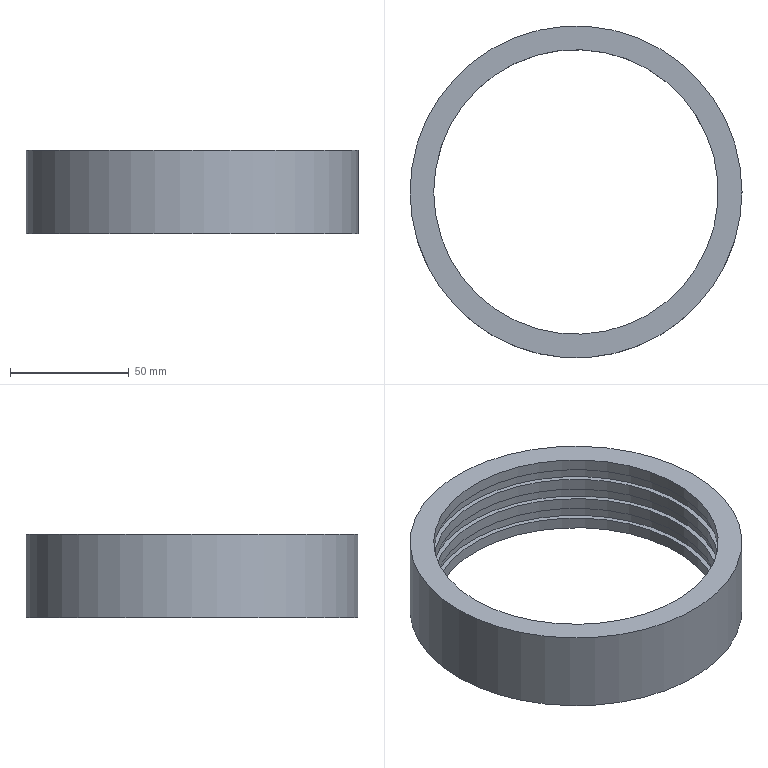Component | NX | CH3404-7 | 1 solid | 16 faces | box 140 x 140 x 35 mm | volume 131444 mm3 | cylinder 8 | plane 8 | commonest cylinder face diameters 120 x4 124 x3 140 x1
STEP:
#1=CARTESIAN_POINT('',(0.,0.,0.));
#2=DIRECTION('',(0.,0.,1.));
#3=DIRECTION('',(1.,0.,0.));
#4=AXIS2_PLACEMENT_3D('',#1,#2,#3);
#5=CARTESIAN_POINT('',(-69.469,0.1057,-1470.003));
#6=VERTEX_POINT('',#5);
#7=CARTESIAN_POINT('',(0.5308,0.1057,-1470.003));
#8=DIRECTION('',(0.,0.,-1.));
#9=DIRECTION('',(-1.,0.,0.));
#10=AXIS2_PLACEMENT_3D('',#7,#8,#9);
#11=CIRCLE('',#10,70.);
#12=CARTESIAN_POINT('',(0.5308,0.1057,-1470.003));
#13=DIRECTION('',(0.,0.,-1.));
#14=DIRECTION('',(-1.,0.,0.));
#15=AXIS2_PLACEMENT_3D('',#12,#13,#14);
#16=CYLINDRICAL_SURFACE('',#15,70.);
#17=CARTESIAN_POINT('',(0.,0.));
#18=DIRECTION('',(1.,0.));
#19=VECTOR('',#18,1.);
#20=LINE('',#17,#19);
#21=(GEOMETRIC_REPRESENTATION_CONTEXT(2)PARAMETRIC_REPRESENTATION_CONTEXT()REPRESENTATION_CONTEXT('',''));
#22=DEFINITIONAL_REPRESENTATION('',(#20),#21);
#23=PCURVE('',#16,#22);
#24=CARTESIAN_POINT('',(0.5308,-69.894,-1470.003));
#25=DIRECTION('',(0.,0.,1.));
#26=DIRECTION('',(1.,0.,0.));
#27=AXIS2_PLACEMENT_3D('',#24,#25,#26);
#28=PLANE('',#27);
#29=CARTESIAN_POINT('',(-70.,70.));
#30=CARTESIAN_POINT('',(-70.,191.244));
#31=CARTESIAN_POINT('',(35.,130.622));
#32=CARTESIAN_POINT('',(140.,70.));
#33=CARTESIAN_POINT('',(35.,9.378));
#34=CARTESIAN_POINT('',(-70.,-51.244));
#35=CARTESIAN_POINT('',(-70.,70.));
#36=(BOUNDED_CURVE()B_SPLINE_CURVE(2,(#29,#30,#31,#32,#33,#34,#35),.UNSPECIFIED.,.T.,.F.)B_SPLINE_CURVE_WITH_KNOTS((1,2,2,2,2,1),(-2.094,0.,2.094,4.189,6.283,8.378),.UNSPECIFIED.)CURVE()GEOMETRIC_REPRESENTATION_ITEM()RATIONAL_B_SPLINE_CURVE((1.,0.5,1.,0.5,1.,0.5,1.))REPRESENTATION_ITEM(''));
#37=(GEOMETRIC_REPRESENTATION_CONTEXT(2)PARAMETRIC_REPRESENTATION_CONTEXT()REPRESENTATION_CONTEXT('',''));
#38=DEFINITIONAL_REPRESENTATION('',(#36),#37);
#39=PCURVE('',#28,#38);
#40=SURFACE_CURVE('',#11,(#23,#39),.PCURVE_S1.);
#41=EDGE_CURVE('',#6,#6,#40,.T.);
#42=ORIENTED_EDGE('',*,*,#41,.F.);
#43=CARTESIAN_POINT('',(-69.469,0.1057,-1435.003));
#44=VERTEX_POINT('',#43);
#45=CARTESIAN_POINT('',(-69.469,0.1057,-1435.003));
#46=CARTESIAN_POINT('',(-69.469,0.1057,-1470.003));
#47=B_SPLINE_CURVE_WITH_KNOTS('',1,(#45,#46),.UNSPECIFIED.,.F.,.F.,(2,2),(-35.,0.),.PIECEWISE_BEZIER_KNOTS.);
#48=CARTESIAN_POINT('',(0.,0.));
#49=DIRECTION('',(0.,1.));
#50=VECTOR('',#49,1.);
#51=LINE('',#48,#50);
#52=(GEOMETRIC_REPRESENTATION_CONTEXT(2)PARAMETRIC_REPRESENTATION_CONTEXT()REPRESENTATION_CONTEXT('',''));
#53=DEFINITIONAL_REPRESENTATION('',(#51),#52);
#54=PCURVE('',#16,#53);
#55=CARTESIAN_POINT('',(6.283,0.));
#56=DIRECTION('',(0.,1.));
#57=VECTOR('',#56,1.);
#58=LINE('',#55,#57);
#59=(GEOMETRIC_REPRESENTATION_CONTEXT(2)PARAMETRIC_REPRESENTATION_CONTEXT()REPRESENTATION_CONTEXT('',''));
#60=DEFINITIONAL_REPRESENTATION('',(#58),#59);
#61=PCURVE('',#16,#60);
#62=SEAM_CURVE('',#47,(#54,#61),.PCURVE_S1.);
#63=EDGE_CURVE('',#44,#6,#62,.T.);
#64=ORIENTED_EDGE('',*,*,#63,.F.);
#65=CARTESIAN_POINT('',(0.5308,0.1057,-1435.003));
#66=DIRECTION('',(0.,0.,-1.));
#67=DIRECTION('',(-1.,0.,0.));
#68=AXIS2_PLACEMENT_3D('',#65,#66,#67);
#69=CIRCLE('',#68,70.);
#70=CARTESIAN_POINT('',(0.,-35.));
#71=DIRECTION('',(1.,0.));
#72=VECTOR('',#71,1.);
#73=LINE('',#70,#72);
#74=(GEOMETRIC_REPRESENTATION_CONTEXT(2)PARAMETRIC_REPRESENTATION_CONTEXT()REPRESENTATION_CONTEXT('',''));
#75=DEFINITIONAL_REPRESENTATION('',(#73),#74);
#76=PCURVE('',#16,#75);
#77=CARTESIAN_POINT('',(0.5308,-59.894,-1435.003));
#78=DIRECTION('',(0.,0.,-1.));
#79=DIRECTION('',(-1.,0.,0.));
#80=AXIS2_PLACEMENT_3D('',#77,#78,#79);
#81=PLANE('',#80);
#82=CARTESIAN_POINT('',(0.,60.));
#83=DIRECTION('',(1.,0.));
#84=AXIS2_PLACEMENT_2D('',#82,#83);
#85=CIRCLE('',#84,70.);
#86=(GEOMETRIC_REPRESENTATION_CONTEXT(2)PARAMETRIC_REPRESENTATION_CONTEXT()REPRESENTATION_CONTEXT('',''));
#87=DEFINITIONAL_REPRESENTATION('',(#85),#86);
#88=PCURVE('',#81,#87);
#89=SURFACE_CURVE('',#69,(#76,#88),.PCURVE_S1.);
#90=EDGE_CURVE('',#44,#44,#89,.T.);
#91=ORIENTED_EDGE('',*,*,#90,.T.);
#92=ORIENTED_EDGE('',*,*,#63,.T.);
#93=EDGE_LOOP('',(#42,#64,#91,#92));
#94=FACE_BOUND('',#93,.T.);
#95=ADVANCED_FACE('',(#94),#16,.T.);
#96=CARTESIAN_POINT('',(-59.469,0.1057,-1470.003));
#97=VERTEX_POINT('',#96);
#98=CARTESIAN_POINT('',(0.5308,0.1057,-1470.003));
#99=DIRECTION('',(0.,0.,-1.));
#100=DIRECTION('',(-1.,0.,0.));
#101=AXIS2_PLACEMENT_3D('',#98,#99,#100);
#102=CIRCLE('',#101,60.);
#103=CARTESIAN_POINT('',(-60.,70.));
#104=CARTESIAN_POINT('',(-60.,173.923));
#105=CARTESIAN_POINT('',(30.,121.962));
#106=CARTESIAN_POINT('',(120.,70.));
#107=CARTESIAN_POINT('',(30.,18.038));
#108=CARTESIAN_POINT('',(-60.,-33.923));
#109=CARTESIAN_POINT('',(-60.,70.));
#110=(BOUNDED_CURVE()B_SPLINE_CURVE(2,(#103,#104,#105,#106,#107,#108,#109),.UNSPECIFIED.,.T.,.F.)B_SPLINE_CURVE_WITH_KNOTS((1,2,2,2,2,1),(-2.094,0.,2.094,4.189,6.283,8.378),.UNSPECIFIED.)CURVE()GEOMETRIC_REPRESENTATION_ITEM()RATIONAL_B_SPLINE_CURVE((1.,0.5,1.,0.5,1.,0.5,1.))REPRESENTATION_ITEM(''));
#111=(GEOMETRIC_REPRESENTATION_CONTEXT(2)PARAMETRIC_REPRESENTATION_CONTEXT()REPRESENTATION_CONTEXT('',''));
#112=DEFINITIONAL_REPRESENTATION('',(#110),#111);
#113=PCURVE('',#28,#112);
#114=CARTESIAN_POINT('',(0.5308,0.1057,-1470.003));
#115=DIRECTION('',(0.,0.,-1.));
#116=DIRECTION('',(-1.,0.,0.));
#117=AXIS2_PLACEMENT_3D('',#114,#115,#116);
#118=CYLINDRICAL_SURFACE('',#117,60.);
#119=CARTESIAN_POINT('',(0.,0.));
#120=DIRECTION('',(1.,0.));
#121=VECTOR('',#120,1.);
#122=LINE('',#119,#121);
#123=(GEOMETRIC_REPRESENTATION_CONTEXT(2)PARAMETRIC_REPRESENTATION_CONTEXT()REPRESENTATION_CONTEXT('',''));
#124=DEFINITIONAL_REPRESENTATION('',(#122),#123);
#125=PCURVE('',#118,#124);
#126=SURFACE_CURVE('',#102,(#113,#125),.PCURVE_S1.);
#127=EDGE_CURVE('',#97,#97,#126,.T.);
#128=ORIENTED_EDGE('',*,*,#127,.F.);
#129=EDGE_LOOP('',(#128));
#130=FACE_BOUND('',#129,.T.);
#131=ORIENTED_EDGE('',*,*,#41,.T.);
#132=EDGE_LOOP('',(#131));
#133=FACE_BOUND('',#132,.T.);
#134=ADVANCED_FACE('',(#130,#133),#28,.F.);
#135=CARTESIAN_POINT('',(-59.469,0.1057,-1465.003));
#136=VERTEX_POINT('',#135);
#137=CARTESIAN_POINT('',(0.5308,0.1057,-1465.003));
#138=DIRECTION('',(0.,0.,-1.));
#139=DIRECTION('',(-1.,0.,0.));
#140=AXIS2_PLACEMENT_3D('',#137,#138,#139);
#141=CIRCLE('',#140,60.);
#142=CARTESIAN_POINT('',(0.,-5.));
#143=DIRECTION('',(1.,0.));
#144=VECTOR('',#143,1.);
#145=LINE('',#142,#144);
#146=(GEOMETRIC_REPRESENTATION_CONTEXT(2)PARAMETRIC_REPRESENTATION_CONTEXT()REPRESENTATION_CONTEXT('',''));
#147=DEFINITIONAL_REPRESENTATION('',(#145),#146);
#148=PCURVE('',#118,#147);
#149=CARTESIAN_POINT('',(0.5308,-59.894,-1465.003));
#150=DIRECTION('',(0.,0.,-1.));
#151=DIRECTION('',(-1.,0.,0.));
#152=AXIS2_PLACEMENT_3D('',#149,#150,#151);
#153=PLANE('',#152);
#154=CARTESIAN_POINT('',(0.,60.));
#155=DIRECTION('',(1.,0.));
#156=AXIS2_PLACEMENT_2D('',#154,#155);
#157=CIRCLE('',#156,60.);
#158=(GEOMETRIC_REPRESENTATION_CONTEXT(2)PARAMETRIC_REPRESENTATION_CONTEXT()REPRESENTATION_CONTEXT('',''));
#159=DEFINITIONAL_REPRESENTATION('',(#157),#158);
#160=PCURVE('',#153,#159);
#161=SURFACE_CURVE('',#141,(#148,#160),.PCURVE_S1.);
#162=EDGE_CURVE('',#136,#136,#161,.T.);
#163=ORIENTED_EDGE('',*,*,#162,.T.);
#164=CARTESIAN_POINT('',(-59.469,0.1057,-1465.003));
#165=CARTESIAN_POINT('',(-59.469,0.1057,-1470.003));
#166=B_SPLINE_CURVE_WITH_KNOTS('',1,(#164,#165),.UNSPECIFIED.,.F.,.F.,(2,2),(-5.,0.),.PIECEWISE_BEZIER_KNOTS.);
#167=CARTESIAN_POINT('',(6.283,0.));
#168=DIRECTION('',(0.,1.));
#169=VECTOR('',#168,1.);
#170=LINE('',#167,#169);
#171=(GEOMETRIC_REPRESENTATION_CONTEXT(2)PARAMETRIC_REPRESENTATION_CONTEXT()REPRESENTATION_CONTEXT('',''));
#172=DEFINITIONAL_REPRESENTATION('',(#170),#171);
#173=PCURVE('',#118,#172);
#174=CARTESIAN_POINT('',(0.,0.));
#175=DIRECTION('',(0.,1.));
#176=VECTOR('',#175,1.);
#177=LINE('',#174,#176);
#178=(GEOMETRIC_REPRESENTATION_CONTEXT(2)PARAMETRIC_REPRESENTATION_CONTEXT()REPRESENTATION_CONTEXT('',''));
#179=DEFINITIONAL_REPRESENTATION('',(#177),#178);
#180=PCURVE('',#118,#179);
#181=SEAM_CURVE('',#166,(#173,#180),.PCURVE_S1.);
#182=EDGE_CURVE('',#136,#97,#181,.T.);
#183=ORIENTED_EDGE('',*,*,#182,.T.);
#184=ORIENTED_EDGE('',*,*,#127,.F.);
#185=ORIENTED_EDGE('',*,*,#182,.F.);
#186=EDGE_LOOP('',(#163,#183,#184,#185));
#187=FACE_BOUND('',#186,.F.);
#188=ADVANCED_FACE('',(#187),#118,.F.);
#189=CARTESIAN_POINT('',(-61.469,0.1057,-1465.003));
#190=VERTEX_POINT('',#189);
#191=CARTESIAN_POINT('',(0.5308,0.1057,-1465.003));
#192=DIRECTION('',(0.,0.,-1.));
#193=DIRECTION('',(-1.,0.,0.));
#194=AXIS2_PLACEMENT_3D('',#191,#192,#193);
#195=CIRCLE('',#194,62.);
#196=CARTESIAN_POINT('',(0.,60.));
#197=DIRECTION('',(1.,0.));
#198=AXIS2_PLACEMENT_2D('',#196,#197);
#199=CIRCLE('',#198,62.);
#200=(GEOMETRIC_REPRESENTATION_CONTEXT(2)PARAMETRIC_REPRESENTATION_CONTEXT()REPRESENTATION_CONTEXT('',''));
#201=DEFINITIONAL_REPRESENTATION('',(#199),#200);
#202=PCURVE('',#153,#201);
#203=CARTESIAN_POINT('',(0.5308,0.1057,-1470.003));
#204=DIRECTION('',(0.,0.,-1.));
#205=DIRECTION('',(-1.,0.,0.));
#206=AXIS2_PLACEMENT_3D('',#203,#204,#205);
#207=CYLINDRICAL_SURFACE('',#206,62.);
#208=CARTESIAN_POINT('',(0.,-5.));
#209=DIRECTION('',(1.,0.));
#210=VECTOR('',#209,1.);
#211=LINE('',#208,#210);
#212=(GEOMETRIC_REPRESENTATION_CONTEXT(2)PARAMETRIC_REPRESENTATION_CONTEXT()REPRESENTATION_CONTEXT('',''));
#213=DEFINITIONAL_REPRESENTATION('',(#211),#212);
#214=PCURVE('',#207,#213);
#215=SURFACE_CURVE('',#195,(#202,#214),.PCURVE_S1.);
#216=EDGE_CURVE('',#190,#190,#215,.T.);
#217=ORIENTED_EDGE('',*,*,#216,.F.);
#218=EDGE_LOOP('',(#217));
#219=FACE_BOUND('',#218,.T.);
#220=ORIENTED_EDGE('',*,*,#162,.T.);
#221=EDGE_LOOP('',(#220));
#222=FACE_BOUND('',#221,.T.);
#223=ADVANCED_FACE('',(#219,#222),#153,.F.);
#224=CARTESIAN_POINT('',(-61.469,0.1057,-1460.003));
#225=VERTEX_POINT('',#224);
#226=CARTESIAN_POINT('',(0.5308,0.1057,-1460.003));
#227=DIRECTION('',(0.,0.,-1.));
#228=DIRECTION('',(-1.,0.,0.));
#229=AXIS2_PLACEMENT_3D('',#226,#227,#228);
#230=CIRCLE('',#229,62.);
#231=CARTESIAN_POINT('',(0.,-10.));
#232=DIRECTION('',(1.,0.));
#233=VECTOR('',#232,1.);
#234=LINE('',#231,#233);
#235=(GEOMETRIC_REPRESENTATION_CONTEXT(2)PARAMETRIC_REPRESENTATION_CONTEXT()REPRESENTATION_CONTEXT('',''));
#236=DEFINITIONAL_REPRESENTATION('',(#234),#235);
#237=PCURVE('',#207,#236);
#238=CARTESIAN_POINT('',(0.5308,-61.894,-1460.003));
#239=DIRECTION('',(0.,0.,1.));
#240=DIRECTION('',(1.,0.,0.));
#241=AXIS2_PLACEMENT_3D('',#238,#239,#240);
#242=PLANE('',#241);
#243=CARTESIAN_POINT('',(-62.,62.));
#244=CARTESIAN_POINT('',(-62.,169.387));
#245=CARTESIAN_POINT('',(31.,115.694));
#246=CARTESIAN_POINT('',(124.,62.));
#247=CARTESIAN_POINT('',(31.,8.306));
#248=CARTESIAN_POINT('',(-62.,-45.387));
#249=CARTESIAN_POINT('',(-62.,62.));
#250=(BOUNDED_CURVE()B_SPLINE_CURVE(2,(#243,#244,#245,#246,#247,#248,#249),.UNSPECIFIED.,.T.,.F.)B_SPLINE_CURVE_WITH_KNOTS((1,2,2,2,2,1),(-2.094,0.,2.094,4.189,6.283,8.378),.UNSPECIFIED.)CURVE()GEOMETRIC_REPRESENTATION_ITEM()RATIONAL_B_SPLINE_CURVE((1.,0.5,1.,0.5,1.,0.5,1.))REPRESENTATION_ITEM(''));
#251=(GEOMETRIC_REPRESENTATION_CONTEXT(2)PARAMETRIC_REPRESENTATION_CONTEXT()REPRESENTATION_CONTEXT('',''));
#252=DEFINITIONAL_REPRESENTATION('',(#250),#251);
#253=PCURVE('',#242,#252);
#254=SURFACE_CURVE('',#230,(#237,#253),.PCURVE_S1.);
#255=EDGE_CURVE('',#225,#225,#254,.T.);
#256=ORIENTED_EDGE('',*,*,#255,.T.);
#257=CARTESIAN_POINT('',(-61.469,0.1057,-1460.003));
#258=CARTESIAN_POINT('',(-61.469,0.1057,-1465.003));
#259=B_SPLINE_CURVE_WITH_KNOTS('',1,(#257,#258),.UNSPECIFIED.,.F.,.F.,(2,2),(-10.,-5.),.PIECEWISE_BEZIER_KNOTS.);
#260=CARTESIAN_POINT('',(6.283,0.));
#261=DIRECTION('',(0.,1.));
#262=VECTOR('',#261,1.);
#263=LINE('',#260,#262);
#264=(GEOMETRIC_REPRESENTATION_CONTEXT(2)PARAMETRIC_REPRESENTATION_CONTEXT()REPRESENTATION_CONTEXT('',''));
#265=DEFINITIONAL_REPRESENTATION('',(#263),#264);
#266=PCURVE('',#207,#265);
#267=CARTESIAN_POINT('',(0.,0.));
#268=DIRECTION('',(0.,1.));
#269=VECTOR('',#268,1.);
#270=LINE('',#267,#269);
#271=(GEOMETRIC_REPRESENTATION_CONTEXT(2)PARAMETRIC_REPRESENTATION_CONTEXT()REPRESENTATION_CONTEXT('',''));
#272=DEFINITIONAL_REPRESENTATION('',(#270),#271);
#273=PCURVE('',#207,#272);
#274=SEAM_CURVE('',#259,(#266,#273),.PCURVE_S1.);
#275=EDGE_CURVE('',#225,#190,#274,.T.);
#276=ORIENTED_EDGE('',*,*,#275,.T.);
#277=ORIENTED_EDGE('',*,*,#216,.F.);
#278=ORIENTED_EDGE('',*,*,#275,.F.);
#279=EDGE_LOOP('',(#256,#276,#277,#278));
#280=FACE_BOUND('',#279,.F.);
#281=ADVANCED_FACE('',(#280),#207,.F.);
#282=CARTESIAN_POINT('',(-59.469,0.1057,-1460.003));
#283=VERTEX_POINT('',#282);
#284=CARTESIAN_POINT('',(0.5308,0.1057,-1460.003));
#285=DIRECTION('',(0.,0.,-1.));
#286=DIRECTION('',(-1.,0.,0.));
#287=AXIS2_PLACEMENT_3D('',#284,#285,#286);
#288=CIRCLE('',#287,60.);
#289=CARTESIAN_POINT('',(-60.,62.));
#290=CARTESIAN_POINT('',(-60.,165.923));
#291=CARTESIAN_POINT('',(30.,113.962));
#292=CARTESIAN_POINT('',(120.,62.));
#293=CARTESIAN_POINT('',(30.,10.038));
#294=CARTESIAN_POINT('',(-60.,-41.923));
#295=CARTESIAN_POINT('',(-60.,62.));
#296=(BOUNDED_CURVE()B_SPLINE_CURVE(2,(#289,#290,#291,#292,#293,#294,#295),.UNSPECIFIED.,.T.,.F.)B_SPLINE_CURVE_WITH_KNOTS((1,2,2,2,2,1),(-2.094,0.,2.094,4.189,6.283,8.378),.UNSPECIFIED.)CURVE()GEOMETRIC_REPRESENTATION_ITEM()RATIONAL_B_SPLINE_CURVE((1.,0.5,1.,0.5,1.,0.5,1.))REPRESENTATION_ITEM(''));
#297=(GEOMETRIC_REPRESENTATION_CONTEXT(2)PARAMETRIC_REPRESENTATION_CONTEXT()REPRESENTATION_CONTEXT('',''));
#298=DEFINITIONAL_REPRESENTATION('',(#296),#297);
#299=PCURVE('',#242,#298);
#300=CARTESIAN_POINT('',(0.5308,0.1057,-1470.003));
#301=DIRECTION('',(0.,0.,-1.));
#302=DIRECTION('',(-1.,0.,0.));
#303=AXIS2_PLACEMENT_3D('',#300,#301,#302);
#304=CYLINDRICAL_SURFACE('',#303,60.);
#305=CARTESIAN_POINT('',(0.,-10.));
#306=DIRECTION('',(1.,0.));
#307=VECTOR('',#306,1.);
#308=LINE('',#305,#307);
#309=(GEOMETRIC_REPRESENTATION_CONTEXT(2)PARAMETRIC_REPRESENTATION_CONTEXT()REPRESENTATION_CONTEXT('',''));
#310=DEFINITIONAL_REPRESENTATION('',(#308),#309);
#311=PCURVE('',#304,#310);
#312=SURFACE_CURVE('',#288,(#299,#311),.PCURVE_S1.);
#313=EDGE_CURVE('',#283,#283,#312,.T.);
#314=ORIENTED_EDGE('',*,*,#313,.F.);
#315=EDGE_LOOP('',(#314));
#316=FACE_BOUND('',#315,.T.);
#317=ORIENTED_EDGE('',*,*,#255,.T.);
#318=EDGE_LOOP('',(#317));
#319=FACE_BOUND('',#318,.T.);
#320=ADVANCED_FACE('',(#316,#319),#242,.F.);
#321=CARTESIAN_POINT('',(-59.469,0.1057,-1455.003));
#322=VERTEX_POINT('',#321);
#323=CARTESIAN_POINT('',(0.5308,0.1057,-1455.003));
#324=DIRECTION('',(0.,0.,-1.));
#325=DIRECTION('',(-1.,0.,0.));
#326=AXIS2_PLACEMENT_3D('',#323,#324,#325);
#327=CIRCLE('',#326,60.);
#328=CARTESIAN_POINT('',(0.,-15.));
#329=DIRECTION('',(1.,0.));
#330=VECTOR('',#329,1.);
#331=LINE('',#328,#330);
#332=(GEOMETRIC_REPRESENTATION_CONTEXT(2)PARAMETRIC_REPRESENTATION_CONTEXT()REPRESENTATION_CONTEXT('',''));
#333=DEFINITIONAL_REPRESENTATION('',(#331),#332);
#334=PCURVE('',#304,#333);
#335=CARTESIAN_POINT('',(0.5308,-59.894,-1455.003));
#336=DIRECTION('',(0.,0.,-1.));
#337=DIRECTION('',(-1.,0.,0.));
#338=AXIS2_PLACEMENT_3D('',#335,#336,#337);
#339=PLANE('',#338);
#340=CARTESIAN_POINT('',(0.,60.));
#341=DIRECTION('',(1.,0.));
#342=AXIS2_PLACEMENT_2D('',#340,#341);
#343=CIRCLE('',#342,60.);
#344=(GEOMETRIC_REPRESENTATION_CONTEXT(2)PARAMETRIC_REPRESENTATION_CONTEXT()REPRESENTATION_CONTEXT('',''));
#345=DEFINITIONAL_REPRESENTATION('',(#343),#344);
#346=PCURVE('',#339,#345);
#347=SURFACE_CURVE('',#327,(#334,#346),.PCURVE_S1.);
#348=EDGE_CURVE('',#322,#322,#347,.T.);
#349=ORIENTED_EDGE('',*,*,#348,.T.);
#350=CARTESIAN_POINT('',(-59.469,0.1057,-1455.003));
#351=CARTESIAN_POINT('',(-59.469,0.1057,-1460.003));
#352=B_SPLINE_CURVE_WITH_KNOTS('',1,(#350,#351),.UNSPECIFIED.,.F.,.F.,(2,2),(-15.,-10.),.PIECEWISE_BEZIER_KNOTS.);
#353=CARTESIAN_POINT('',(6.283,0.));
#354=DIRECTION('',(0.,1.));
#355=VECTOR('',#354,1.);
#356=LINE('',#353,#355);
#357=(GEOMETRIC_REPRESENTATION_CONTEXT(2)PARAMETRIC_REPRESENTATION_CONTEXT()REPRESENTATION_CONTEXT('',''));
#358=DEFINITIONAL_REPRESENTATION('',(#356),#357);
#359=PCURVE('',#304,#358);
#360=CARTESIAN_POINT('',(0.,0.));
#361=DIRECTION('',(0.,1.));
#362=VECTOR('',#361,1.);
#363=LINE('',#360,#362);
#364=(GEOMETRIC_REPRESENTATION_CONTEXT(2)PARAMETRIC_REPRESENTATION_CONTEXT()REPRESENTATION_CONTEXT('',''));
#365=DEFINITIONAL_REPRESENTATION('',(#363),#364);
#366=PCURVE('',#304,#365);
#367=SEAM_CURVE('',#352,(#359,#366),.PCURVE_S1.);
#368=EDGE_CURVE('',#322,#283,#367,.T.);
#369=ORIENTED_EDGE('',*,*,#368,.T.);
#370=ORIENTED_EDGE('',*,*,#313,.F.);
#371=ORIENTED_EDGE('',*,*,#368,.F.);
#372=EDGE_LOOP('',(#349,#369,#370,#371));
#373=FACE_BOUND('',#372,.F.);
#374=ADVANCED_FACE('',(#373),#304,.F.);
#375=CARTESIAN_POINT('',(-61.469,0.1057,-1455.003));
#376=VERTEX_POINT('',#375);
#377=CARTESIAN_POINT('',(0.5308,0.1057,-1455.003));
#378=DIRECTION('',(0.,0.,-1.));
#379=DIRECTION('',(-1.,0.,0.));
#380=AXIS2_PLACEMENT_3D('',#377,#378,#379);
#381=CIRCLE('',#380,62.);
#382=CARTESIAN_POINT('',(0.,60.));
#383=DIRECTION('',(1.,0.));
#384=AXIS2_PLACEMENT_2D('',#382,#383);
#385=CIRCLE('',#384,62.);
#386=(GEOMETRIC_REPRESENTATION_CONTEXT(2)PARAMETRIC_REPRESENTATION_CONTEXT()REPRESENTATION_CONTEXT('',''));
#387=DEFINITIONAL_REPRESENTATION('',(#385),#386);
#388=PCURVE('',#339,#387);
#389=CARTESIAN_POINT('',(0.5308,0.1057,-1470.003));
#390=DIRECTION('',(0.,0.,-1.));
#391=DIRECTION('',(-1.,0.,0.));
#392=AXIS2_PLACEMENT_3D('',#389,#390,#391);
#393=CYLINDRICAL_SURFACE('',#392,62.);
#394=CARTESIAN_POINT('',(0.,-15.));
#395=DIRECTION('',(1.,0.));
#396=VECTOR('',#395,1.);
#397=LINE('',#394,#396);
#398=(GEOMETRIC_REPRESENTATION_CONTEXT(2)PARAMETRIC_REPRESENTATION_CONTEXT()REPRESENTATION_CONTEXT('',''));
#399=DEFINITIONAL_REPRESENTATION('',(#397),#398);
#400=PCURVE('',#393,#399);
#401=SURFACE_CURVE('',#381,(#388,#400),.PCURVE_S1.);
#402=EDGE_CURVE('',#376,#376,#401,.T.);
#403=ORIENTED_EDGE('',*,*,#402,.F.);
#404=EDGE_LOOP('',(#403));
#405=FACE_BOUND('',#404,.T.);
#406=ORIENTED_EDGE('',*,*,#348,.T.);
#407=EDGE_LOOP('',(#406));
#408=FACE_BOUND('',#407,.T.);
#409=ADVANCED_FACE('',(#405,#408),#339,.F.);
#410=CARTESIAN_POINT('',(-61.469,0.1057,-1450.003));
#411=VERTEX_POINT('',#410);
#412=CARTESIAN_POINT('',(0.5308,0.1057,-1450.003));
#413=DIRECTION('',(0.,0.,-1.));
#414=DIRECTION('',(-1.,0.,0.));
#415=AXIS2_PLACEMENT_3D('',#412,#413,#414);
#416=CIRCLE('',#415,62.);
#417=CARTESIAN_POINT('',(0.,-20.));
#418=DIRECTION('',(1.,0.));
#419=VECTOR('',#418,1.);
#420=LINE('',#417,#419);
#421=(GEOMETRIC_REPRESENTATION_CONTEXT(2)PARAMETRIC_REPRESENTATION_CONTEXT()REPRESENTATION_CONTEXT('',''));
#422=DEFINITIONAL_REPRESENTATION('',(#420),#421);
#423=PCURVE('',#393,#422);
#424=CARTESIAN_POINT('',(0.5308,-61.894,-1450.003));
#425=DIRECTION('',(0.,0.,1.));
#426=DIRECTION('',(1.,0.,0.));
#427=AXIS2_PLACEMENT_3D('',#424,#425,#426);
#428=PLANE('',#427);
#429=CARTESIAN_POINT('',(-62.,62.));
#430=CARTESIAN_POINT('',(-62.,169.387));
#431=CARTESIAN_POINT('',(31.,115.694));
#432=CARTESIAN_POINT('',(124.,62.));
#433=CARTESIAN_POINT('',(31.,8.306));
#434=CARTESIAN_POINT('',(-62.,-45.387));
#435=CARTESIAN_POINT('',(-62.,62.));
#436=(BOUNDED_CURVE()B_SPLINE_CURVE(2,(#429,#430,#431,#432,#433,#434,#435),.UNSPECIFIED.,.T.,.F.)B_SPLINE_CURVE_WITH_KNOTS((1,2,2,2,2,1),(-2.094,0.,2.094,4.189,6.283,8.378),.UNSPECIFIED.)CURVE()GEOMETRIC_REPRESENTATION_ITEM()RATIONAL_B_SPLINE_CURVE((1.,0.5,1.,0.5,1.,0.5,1.))REPRESENTATION_ITEM(''));
#437=(GEOMETRIC_REPRESENTATION_CONTEXT(2)PARAMETRIC_REPRESENTATION_CONTEXT()REPRESENTATION_CONTEXT('',''));
#438=DEFINITIONAL_REPRESENTATION('',(#436),#437);
#439=PCURVE('',#428,#438);
#440=SURFACE_CURVE('',#416,(#423,#439),.PCURVE_S1.);
#441=EDGE_CURVE('',#411,#411,#440,.T.);
#442=ORIENTED_EDGE('',*,*,#441,.T.);
#443=CARTESIAN_POINT('',(-61.469,0.1057,-1450.003));
#444=CARTESIAN_POINT('',(-61.469,0.1057,-1455.003));
#445=B_SPLINE_CURVE_WITH_KNOTS('',1,(#443,#444),.UNSPECIFIED.,.F.,.F.,(2,2),(-20.,-15.),.PIECEWISE_BEZIER_KNOTS.);
#446=CARTESIAN_POINT('',(6.283,0.));
#447=DIRECTION('',(0.,1.));
#448=VECTOR('',#447,1.);
#449=LINE('',#446,#448);
#450=(GEOMETRIC_REPRESENTATION_CONTEXT(2)PARAMETRIC_REPRESENTATION_CONTEXT()REPRESENTATION_CONTEXT('',''));
#451=DEFINITIONAL_REPRESENTATION('',(#449),#450);
#452=PCURVE('',#393,#451);
#453=CARTESIAN_POINT('',(0.,0.));
#454=DIRECTION('',(0.,1.));
#455=VECTOR('',#454,1.);
#456=LINE('',#453,#455);
#457=(GEOMETRIC_REPRESENTATION_CONTEXT(2)PARAMETRIC_REPRESENTATION_CONTEXT()REPRESENTATION_CONTEXT('',''));
#458=DEFINITIONAL_REPRESENTATION('',(#456),#457);
#459=PCURVE('',#393,#458);
#460=SEAM_CURVE('',#445,(#452,#459),.PCURVE_S1.);
#461=EDGE_CURVE('',#411,#376,#460,.T.);
#462=ORIENTED_EDGE('',*,*,#461,.T.);
#463=ORIENTED_EDGE('',*,*,#402,.F.);
#464=ORIENTED_EDGE('',*,*,#461,.F.);
#465=EDGE_LOOP('',(#442,#462,#463,#464));
#466=FACE_BOUND('',#465,.F.);
#467=ADVANCED_FACE('',(#466),#393,.F.);
#468=CARTESIAN_POINT('',(-59.469,0.1057,-1450.003));
#469=VERTEX_POINT('',#468);
#470=CARTESIAN_POINT('',(0.5308,0.1057,-1450.003));
#471=DIRECTION('',(0.,0.,-1.));
#472=DIRECTION('',(-1.,0.,0.));
#473=AXIS2_PLACEMENT_3D('',#470,#471,#472);
#474=CIRCLE('',#473,60.);
#475=CARTESIAN_POINT('',(-60.,62.));
#476=CARTESIAN_POINT('',(-60.,165.923));
#477=CARTESIAN_POINT('',(30.,113.962));
#478=CARTESIAN_POINT('',(120.,62.));
#479=CARTESIAN_POINT('',(30.,10.038));
#480=CARTESIAN_POINT('',(-60.,-41.923));
#481=CARTESIAN_POINT('',(-60.,62.));
#482=(BOUNDED_CURVE()B_SPLINE_CURVE(2,(#475,#476,#477,#478,#479,#480,#481),.UNSPECIFIED.,.T.,.F.)B_SPLINE_CURVE_WITH_KNOTS((1,2,2,2,2,1),(-2.094,0.,2.094,4.189,6.283,8.378),.UNSPECIFIED.)CURVE()GEOMETRIC_REPRESENTATION_ITEM()RATIONAL_B_SPLINE_CURVE((1.,0.5,1.,0.5,1.,0.5,1.))REPRESENTATION_ITEM(''));
#483=(GEOMETRIC_REPRESENTATION_CONTEXT(2)PARAMETRIC_REPRESENTATION_CONTEXT()REPRESENTATION_CONTEXT('',''));
#484=DEFINITIONAL_REPRESENTATION('',(#482),#483);
#485=PCURVE('',#428,#484);
#486=CARTESIAN_POINT('',(0.5308,0.1057,-1470.003));
#487=DIRECTION('',(0.,0.,-1.));
#488=DIRECTION('',(-1.,0.,0.));
#489=AXIS2_PLACEMENT_3D('',#486,#487,#488);
#490=CYLINDRICAL_SURFACE('',#489,60.);
#491=CARTESIAN_POINT('',(0.,-20.));
#492=DIRECTION('',(1.,0.));
#493=VECTOR('',#492,1.);
#494=LINE('',#491,#493);
#495=(GEOMETRIC_REPRESENTATION_CONTEXT(2)PARAMETRIC_REPRESENTATION_CONTEXT()REPRESENTATION_CONTEXT('',''));
#496=DEFINITIONAL_REPRESENTATION('',(#494),#495);
#497=PCURVE('',#490,#496);
#498=SURFACE_CURVE('',#474,(#485,#497),.PCURVE_S1.);
#499=EDGE_CURVE('',#469,#469,#498,.T.);
#500=ORIENTED_EDGE('',*,*,#499,.F.);
#501=EDGE_LOOP('',(#500));
#502=FACE_BOUND('',#501,.T.);
#503=ORIENTED_EDGE('',*,*,#441,.T.);
#504=EDGE_LOOP('',(#503));
#505=FACE_BOUND('',#504,.T.);
#506=ADVANCED_FACE('',(#502,#505),#428,.F.);
#507=CARTESIAN_POINT('',(-59.469,0.1057,-1445.003));
#508=VERTEX_POINT('',#507);
#509=CARTESIAN_POINT('',(0.5308,0.1057,-1445.003));
#510=DIRECTION('',(0.,0.,-1.));
#511=DIRECTION('',(-1.,0.,0.));
#512=AXIS2_PLACEMENT_3D('',#509,#510,#511);
#513=CIRCLE('',#512,60.);
#514=CARTESIAN_POINT('',(0.,-25.));
#515=DIRECTION('',(1.,0.));
#516=VECTOR('',#515,1.);
#517=LINE('',#514,#516);
#518=(GEOMETRIC_REPRESENTATION_CONTEXT(2)PARAMETRIC_REPRESENTATION_CONTEXT()REPRESENTATION_CONTEXT('',''));
#519=DEFINITIONAL_REPRESENTATION('',(#517),#518);
#520=PCURVE('',#490,#519);
#521=CARTESIAN_POINT('',(0.5308,-59.894,-1445.003));
#522=DIRECTION('',(0.,0.,-1.));
#523=DIRECTION('',(-1.,0.,0.));
#524=AXIS2_PLACEMENT_3D('',#521,#522,#523);
#525=PLANE('',#524);
#526=CARTESIAN_POINT('',(0.,60.));
#527=DIRECTION('',(1.,0.));
#528=AXIS2_PLACEMENT_2D('',#526,#527);
#529=CIRCLE('',#528,60.);
#530=(GEOMETRIC_REPRESENTATION_CONTEXT(2)PARAMETRIC_REPRESENTATION_CONTEXT()REPRESENTATION_CONTEXT('',''));
#531=DEFINITIONAL_REPRESENTATION('',(#529),#530);
#532=PCURVE('',#525,#531);
#533=SURFACE_CURVE('',#513,(#520,#532),.PCURVE_S1.);
#534=EDGE_CURVE('',#508,#508,#533,.T.);
#535=ORIENTED_EDGE('',*,*,#534,.T.);
#536=CARTESIAN_POINT('',(-59.469,0.1057,-1445.003));
#537=CARTESIAN_POINT('',(-59.469,0.1057,-1450.003));
#538=B_SPLINE_CURVE_WITH_KNOTS('',1,(#536,#537),.UNSPECIFIED.,.F.,.F.,(2,2),(-25.,-20.),.PIECEWISE_BEZIER_KNOTS.);
#539=CARTESIAN_POINT('',(6.283,0.));
#540=DIRECTION('',(0.,1.));
#541=VECTOR('',#540,1.);
#542=LINE('',#539,#541);
#543=(GEOMETRIC_REPRESENTATION_CONTEXT(2)PARAMETRIC_REPRESENTATION_CONTEXT()REPRESENTATION_CONTEXT('',''));
#544=DEFINITIONAL_REPRESENTATION('',(#542),#543);
#545=PCURVE('',#490,#544);
#546=CARTESIAN_POINT('',(0.,0.));
#547=DIRECTION('',(0.,1.));
#548=VECTOR('',#547,1.);
#549=LINE('',#546,#548);
#550=(GEOMETRIC_REPRESENTATION_CONTEXT(2)PARAMETRIC_REPRESENTATION_CONTEXT()REPRESENTATION_CONTEXT('',''));
#551=DEFINITIONAL_REPRESENTATION('',(#549),#550);
#552=PCURVE('',#490,#551);
#553=SEAM_CURVE('',#538,(#545,#552),.PCURVE_S1.);
#554=EDGE_CURVE('',#508,#469,#553,.T.);
#555=ORIENTED_EDGE('',*,*,#554,.T.);
#556=ORIENTED_EDGE('',*,*,#499,.F.);
#557=ORIENTED_EDGE('',*,*,#554,.F.);
#558=EDGE_LOOP('',(#535,#555,#556,#557));
#559=FACE_BOUND('',#558,.F.);
#560=ADVANCED_FACE('',(#559),#490,.F.);
#561=CARTESIAN_POINT('',(-61.469,0.1057,-1445.003));
#562=VERTEX_POINT('',#561);
#563=CARTESIAN_POINT('',(0.5308,0.1057,-1445.003));
#564=DIRECTION('',(0.,0.,-1.));
#565=DIRECTION('',(-1.,0.,0.));
#566=AXIS2_PLACEMENT_3D('',#563,#564,#565);
#567=CIRCLE('',#566,62.);
#568=CARTESIAN_POINT('',(0.,60.));
#569=DIRECTION('',(1.,0.));
#570=AXIS2_PLACEMENT_2D('',#568,#569);
#571=CIRCLE('',#570,62.);
#572=(GEOMETRIC_REPRESENTATION_CONTEXT(2)PARAMETRIC_REPRESENTATION_CONTEXT()REPRESENTATION_CONTEXT('',''));
#573=DEFINITIONAL_REPRESENTATION('',(#571),#572);
#574=PCURVE('',#525,#573);
#575=CARTESIAN_POINT('',(0.5308,0.1057,-1470.003));
#576=DIRECTION('',(0.,0.,-1.));
#577=DIRECTION('',(-1.,0.,0.));
#578=AXIS2_PLACEMENT_3D('',#575,#576,#577);
#579=CYLINDRICAL_SURFACE('',#578,62.);
#580=CARTESIAN_POINT('',(0.,-25.));
#581=DIRECTION('',(1.,0.));
#582=VECTOR('',#581,1.);
#583=LINE('',#580,#582);
#584=(GEOMETRIC_REPRESENTATION_CONTEXT(2)PARAMETRIC_REPRESENTATION_CONTEXT()REPRESENTATION_CONTEXT('',''));
#585=DEFINITIONAL_REPRESENTATION('',(#583),#584);
#586=PCURVE('',#579,#585);
#587=SURFACE_CURVE('',#567,(#574,#586),.PCURVE_S1.);
#588=EDGE_CURVE('',#562,#562,#587,.T.);
#589=ORIENTED_EDGE('',*,*,#588,.F.);
#590=EDGE_LOOP('',(#589));
#591=FACE_BOUND('',#590,.T.);
#592=ORIENTED_EDGE('',*,*,#534,.T.);
#593=EDGE_LOOP('',(#592));
#594=FACE_BOUND('',#593,.T.);
#595=ADVANCED_FACE('',(#591,#594),#525,.F.);
#596=CARTESIAN_POINT('',(-61.469,0.1057,-1440.003));
#597=VERTEX_POINT('',#596);
#598=CARTESIAN_POINT('',(0.5308,0.1057,-1440.003));
#599=DIRECTION('',(0.,0.,-1.));
#600=DIRECTION('',(-1.,0.,0.));
#601=AXIS2_PLACEMENT_3D('',#598,#599,#600);
#602=CIRCLE('',#601,62.);
#603=CARTESIAN_POINT('',(0.,-30.));
#604=DIRECTION('',(1.,0.));
#605=VECTOR('',#604,1.);
#606=LINE('',#603,#605);
#607=(GEOMETRIC_REPRESENTATION_CONTEXT(2)PARAMETRIC_REPRESENTATION_CONTEXT()REPRESENTATION_CONTEXT('',''));
#608=DEFINITIONAL_REPRESENTATION('',(#606),#607);
#609=PCURVE('',#579,#608);
#610=CARTESIAN_POINT('',(0.5308,-61.894,-1440.003));
#611=DIRECTION('',(0.,0.,1.));
#612=DIRECTION('',(1.,0.,0.));
#613=AXIS2_PLACEMENT_3D('',#610,#611,#612);
#614=PLANE('',#613);
#615=CARTESIAN_POINT('',(-62.,62.));
#616=CARTESIAN_POINT('',(-62.,169.387));
#617=CARTESIAN_POINT('',(31.,115.694));
#618=CARTESIAN_POINT('',(124.,62.));
#619=CARTESIAN_POINT('',(31.,8.306));
#620=CARTESIAN_POINT('',(-62.,-45.387));
#621=CARTESIAN_POINT('',(-62.,62.));
#622=(BOUNDED_CURVE()B_SPLINE_CURVE(2,(#615,#616,#617,#618,#619,#620,#621),.UNSPECIFIED.,.T.,.F.)B_SPLINE_CURVE_WITH_KNOTS((1,2,2,2,2,1),(-2.094,0.,2.094,4.189,6.283,8.378),.UNSPECIFIED.)CURVE()GEOMETRIC_REPRESENTATION_ITEM()RATIONAL_B_SPLINE_CURVE((1.,0.5,1.,0.5,1.,0.5,1.))REPRESENTATION_ITEM(''));
#623=(GEOMETRIC_REPRESENTATION_CONTEXT(2)PARAMETRIC_REPRESENTATION_CONTEXT()REPRESENTATION_CONTEXT('',''));
#624=DEFINITIONAL_REPRESENTATION('',(#622),#623);
#625=PCURVE('',#614,#624);
#626=SURFACE_CURVE('',#602,(#609,#625),.PCURVE_S1.);
#627=EDGE_CURVE('',#597,#597,#626,.T.);
#628=ORIENTED_EDGE('',*,*,#627,.T.);
#629=CARTESIAN_POINT('',(-61.469,0.1057,-1440.003));
#630=CARTESIAN_POINT('',(-61.469,0.1057,-1445.003));
#631=B_SPLINE_CURVE_WITH_KNOTS('',1,(#629,#630),.UNSPECIFIED.,.F.,.F.,(2,2),(-30.,-25.),.PIECEWISE_BEZIER_KNOTS.);
#632=CARTESIAN_POINT('',(6.283,0.));
#633=DIRECTION('',(0.,1.));
#634=VECTOR('',#633,1.);
#635=LINE('',#632,#634);
#636=(GEOMETRIC_REPRESENTATION_CONTEXT(2)PARAMETRIC_REPRESENTATION_CONTEXT()REPRESENTATION_CONTEXT('',''));
#637=DEFINITIONAL_REPRESENTATION('',(#635),#636);
#638=PCURVE('',#579,#637);
#639=CARTESIAN_POINT('',(0.,0.));
#640=DIRECTION('',(0.,1.));
#641=VECTOR('',#640,1.);
#642=LINE('',#639,#641);
#643=(GEOMETRIC_REPRESENTATION_CONTEXT(2)PARAMETRIC_REPRESENTATION_CONTEXT()REPRESENTATION_CONTEXT('',''));
#644=DEFINITIONAL_REPRESENTATION('',(#642),#643);
#645=PCURVE('',#579,#644);
#646=SEAM_CURVE('',#631,(#638,#645),.PCURVE_S1.);
#647=EDGE_CURVE('',#597,#562,#646,.T.);
#648=ORIENTED_EDGE('',*,*,#647,.T.);
#649=ORIENTED_EDGE('',*,*,#588,.F.);
#650=ORIENTED_EDGE('',*,*,#647,.F.);
#651=EDGE_LOOP('',(#628,#648,#649,#650));
#652=FACE_BOUND('',#651,.F.);
#653=ADVANCED_FACE('',(#652),#579,.F.);
#654=CARTESIAN_POINT('',(-59.469,0.1057,-1440.003));
#655=VERTEX_POINT('',#654);
#656=CARTESIAN_POINT('',(0.5308,0.1057,-1440.003));
#657=DIRECTION('',(0.,0.,-1.));
#658=DIRECTION('',(-1.,0.,0.));
#659=AXIS2_PLACEMENT_3D('',#656,#657,#658);
#660=CIRCLE('',#659,60.);
#661=CARTESIAN_POINT('',(-60.,62.));
#662=CARTESIAN_POINT('',(-60.,165.923));
#663=CARTESIAN_POINT('',(30.,113.962));
#664=CARTESIAN_POINT('',(120.,62.));
#665=CARTESIAN_POINT('',(30.,10.038));
#666=CARTESIAN_POINT('',(-60.,-41.923));
#667=CARTESIAN_POINT('',(-60.,62.));
#668=(BOUNDED_CURVE()B_SPLINE_CURVE(2,(#661,#662,#663,#664,#665,#666,#667),.UNSPECIFIED.,.T.,.F.)B_SPLINE_CURVE_WITH_KNOTS((1,2,2,2,2,1),(-2.094,0.,2.094,4.189,6.283,8.378),.UNSPECIFIED.)CURVE()GEOMETRIC_REPRESENTATION_ITEM()RATIONAL_B_SPLINE_CURVE((1.,0.5,1.,0.5,1.,0.5,1.))REPRESENTATION_ITEM(''));
#669=(GEOMETRIC_REPRESENTATION_CONTEXT(2)PARAMETRIC_REPRESENTATION_CONTEXT()REPRESENTATION_CONTEXT('',''));
#670=DEFINITIONAL_REPRESENTATION('',(#668),#669);
#671=PCURVE('',#614,#670);
#672=CARTESIAN_POINT('',(0.5308,0.1057,-1470.003));
#673=DIRECTION('',(0.,0.,-1.));
#674=DIRECTION('',(-1.,0.,0.));
#675=AXIS2_PLACEMENT_3D('',#672,#673,#674);
#676=CYLINDRICAL_SURFACE('',#675,60.);
#677=CARTESIAN_POINT('',(0.,-30.));
#678=DIRECTION('',(1.,0.));
#679=VECTOR('',#678,1.);
#680=LINE('',#677,#679);
#681=(GEOMETRIC_REPRESENTATION_CONTEXT(2)PARAMETRIC_REPRESENTATION_CONTEXT()REPRESENTATION_CONTEXT('',''));
#682=DEFINITIONAL_REPRESENTATION('',(#680),#681);
#683=PCURVE('',#676,#682);
#684=SURFACE_CURVE('',#660,(#671,#683),.PCURVE_S1.);
#685=EDGE_CURVE('',#655,#655,#684,.T.);
#686=ORIENTED_EDGE('',*,*,#685,.F.);
#687=EDGE_LOOP('',(#686));
#688=FACE_BOUND('',#687,.T.);
#689=ORIENTED_EDGE('',*,*,#627,.T.);
#690=EDGE_LOOP('',(#689));
#691=FACE_BOUND('',#690,.T.);
#692=ADVANCED_FACE('',(#688,#691),#614,.F.);
#693=CARTESIAN_POINT('',(-59.469,0.1057,-1435.003));
#694=VERTEX_POINT('',#693);
#695=CARTESIAN_POINT('',(0.5308,0.1057,-1435.003));
#696=DIRECTION('',(0.,0.,-1.));
#697=DIRECTION('',(-1.,0.,0.));
#698=AXIS2_PLACEMENT_3D('',#695,#696,#697);
#699=CIRCLE('',#698,60.);
#700=CARTESIAN_POINT('',(0.,-35.));
#701=DIRECTION('',(1.,0.));
#702=VECTOR('',#701,1.);
#703=LINE('',#700,#702);
#704=(GEOMETRIC_REPRESENTATION_CONTEXT(2)PARAMETRIC_REPRESENTATION_CONTEXT()REPRESENTATION_CONTEXT('',''));
#705=DEFINITIONAL_REPRESENTATION('',(#703),#704);
#706=PCURVE('',#676,#705);
#707=CARTESIAN_POINT('',(0.,60.));
#708=DIRECTION('',(1.,0.));
#709=AXIS2_PLACEMENT_2D('',#707,#708);
#710=CIRCLE('',#709,60.);
#711=(GEOMETRIC_REPRESENTATION_CONTEXT(2)PARAMETRIC_REPRESENTATION_CONTEXT()REPRESENTATION_CONTEXT('',''));
#712=DEFINITIONAL_REPRESENTATION('',(#710),#711);
#713=PCURVE('',#81,#712);
#714=SURFACE_CURVE('',#699,(#706,#713),.PCURVE_S1.);
#715=EDGE_CURVE('',#694,#694,#714,.T.);
#716=ORIENTED_EDGE('',*,*,#715,.T.);
#717=CARTESIAN_POINT('',(-59.469,0.1057,-1435.003));
#718=CARTESIAN_POINT('',(-59.469,0.1057,-1440.003));
#719=B_SPLINE_CURVE_WITH_KNOTS('',1,(#717,#718),.UNSPECIFIED.,.F.,.F.,(2,2),(-35.,-30.),.PIECEWISE_BEZIER_KNOTS.);
#720=CARTESIAN_POINT('',(6.283,0.));
#721=DIRECTION('',(0.,1.));
#722=VECTOR('',#721,1.);
#723=LINE('',#720,#722);
#724=(GEOMETRIC_REPRESENTATION_CONTEXT(2)PARAMETRIC_REPRESENTATION_CONTEXT()REPRESENTATION_CONTEXT('',''));
#725=DEFINITIONAL_REPRESENTATION('',(#723),#724);
#726=PCURVE('',#676,#725);
#727=CARTESIAN_POINT('',(0.,0.));
#728=DIRECTION('',(0.,1.));
#729=VECTOR('',#728,1.);
#730=LINE('',#727,#729);
#731=(GEOMETRIC_REPRESENTATION_CONTEXT(2)PARAMETRIC_REPRESENTATION_CONTEXT()REPRESENTATION_CONTEXT('',''));
#732=DEFINITIONAL_REPRESENTATION('',(#730),#731);
#733=PCURVE('',#676,#732);
#734=SEAM_CURVE('',#719,(#726,#733),.PCURVE_S1.);
#735=EDGE_CURVE('',#694,#655,#734,.T.);
#736=ORIENTED_EDGE('',*,*,#735,.T.);
#737=ORIENTED_EDGE('',*,*,#685,.F.);
#738=ORIENTED_EDGE('',*,*,#735,.F.);
#739=EDGE_LOOP('',(#716,#736,#737,#738));
#740=FACE_BOUND('',#739,.F.);
#741=ADVANCED_FACE('',(#740),#676,.F.);
#742=ORIENTED_EDGE('',*,*,#90,.F.);
#743=EDGE_LOOP('',(#742));
#744=FACE_BOUND('',#743,.T.);
#745=ORIENTED_EDGE('',*,*,#715,.T.);
#746=EDGE_LOOP('',(#745));
#747=FACE_BOUND('',#746,.T.);
#748=ADVANCED_FACE('',(#744,#747),#81,.F.);
#749=CLOSED_SHELL('',(#95,#134,#188,#223,#281,#320,#374,#409,#467,#506,#560,#595,#653,#692,#741,#748));
#750=MANIFOLD_SOLID_BREP('',#749);
#751=(LENGTH_UNIT()NAMED_UNIT(*)SI_UNIT(.MILLI.,.METRE.));
#752=UNCERTAINTY_MEASURE_WITH_UNIT(LENGTH_MEASURE(0.00001),#751,'','');
#753=(NAMED_UNIT(*)PLANE_ANGLE_UNIT()SI_UNIT($,.RADIAN.));
#754=(NAMED_UNIT(*)SI_UNIT($,.STERADIAN.)SOLID_ANGLE_UNIT());
#755=(GEOMETRIC_REPRESENTATION_CONTEXT(3)GLOBAL_UNCERTAINTY_ASSIGNED_CONTEXT((#752))GLOBAL_UNIT_ASSIGNED_CONTEXT((#751,#753,#754))REPRESENTATION_CONTEXT('',''));
#756=ADVANCED_BREP_SHAPE_REPRESENTATION('',(#4,#750),#755);